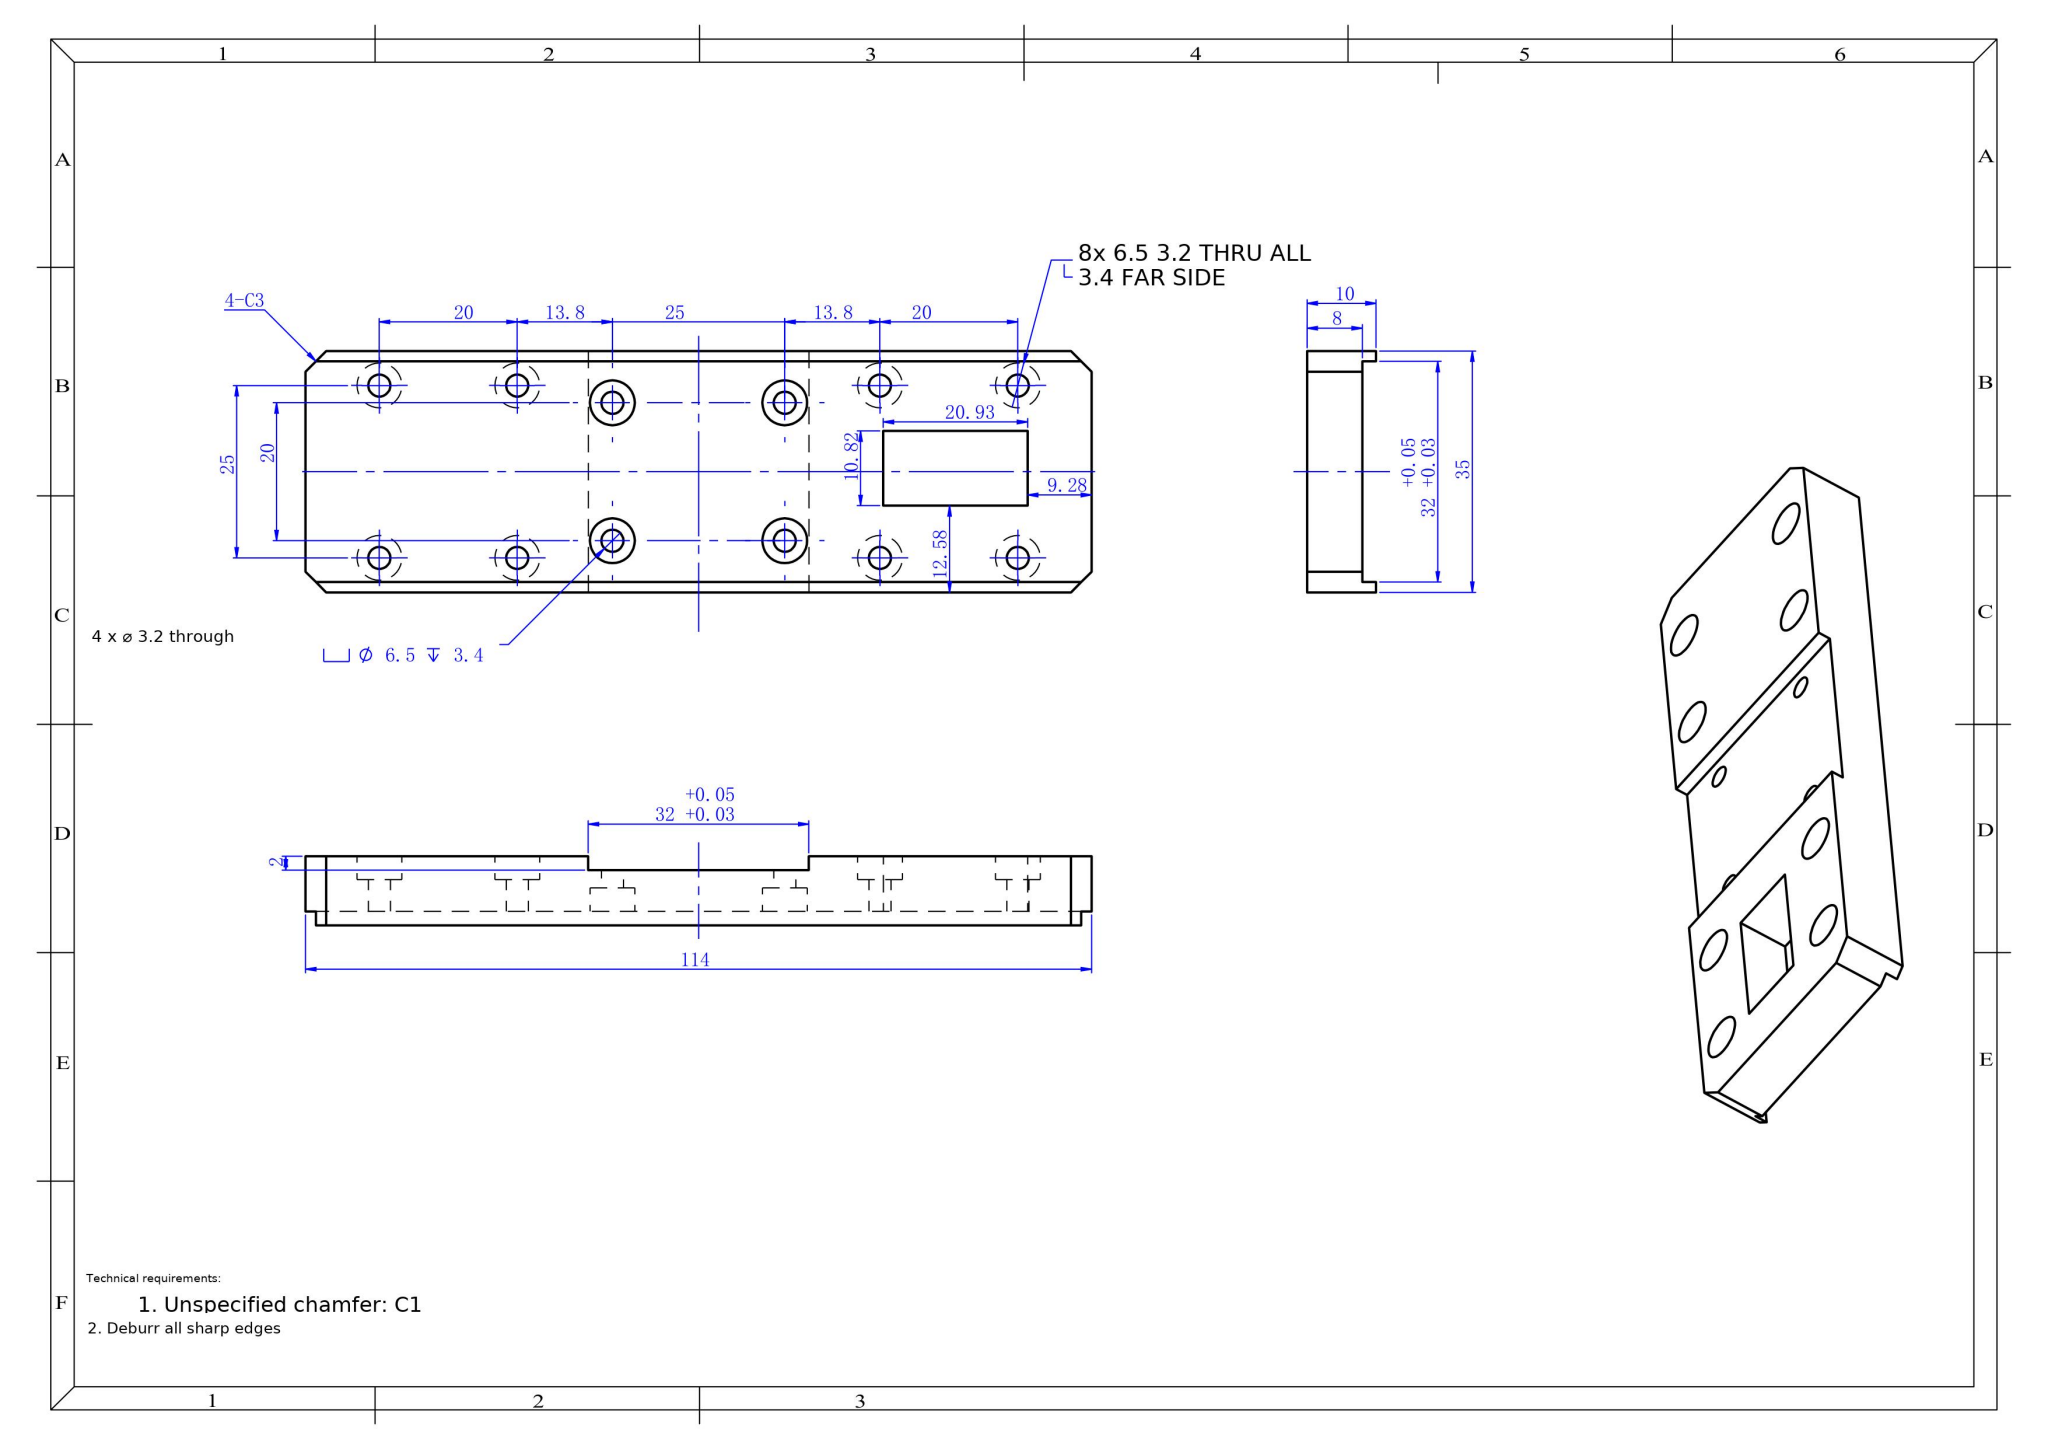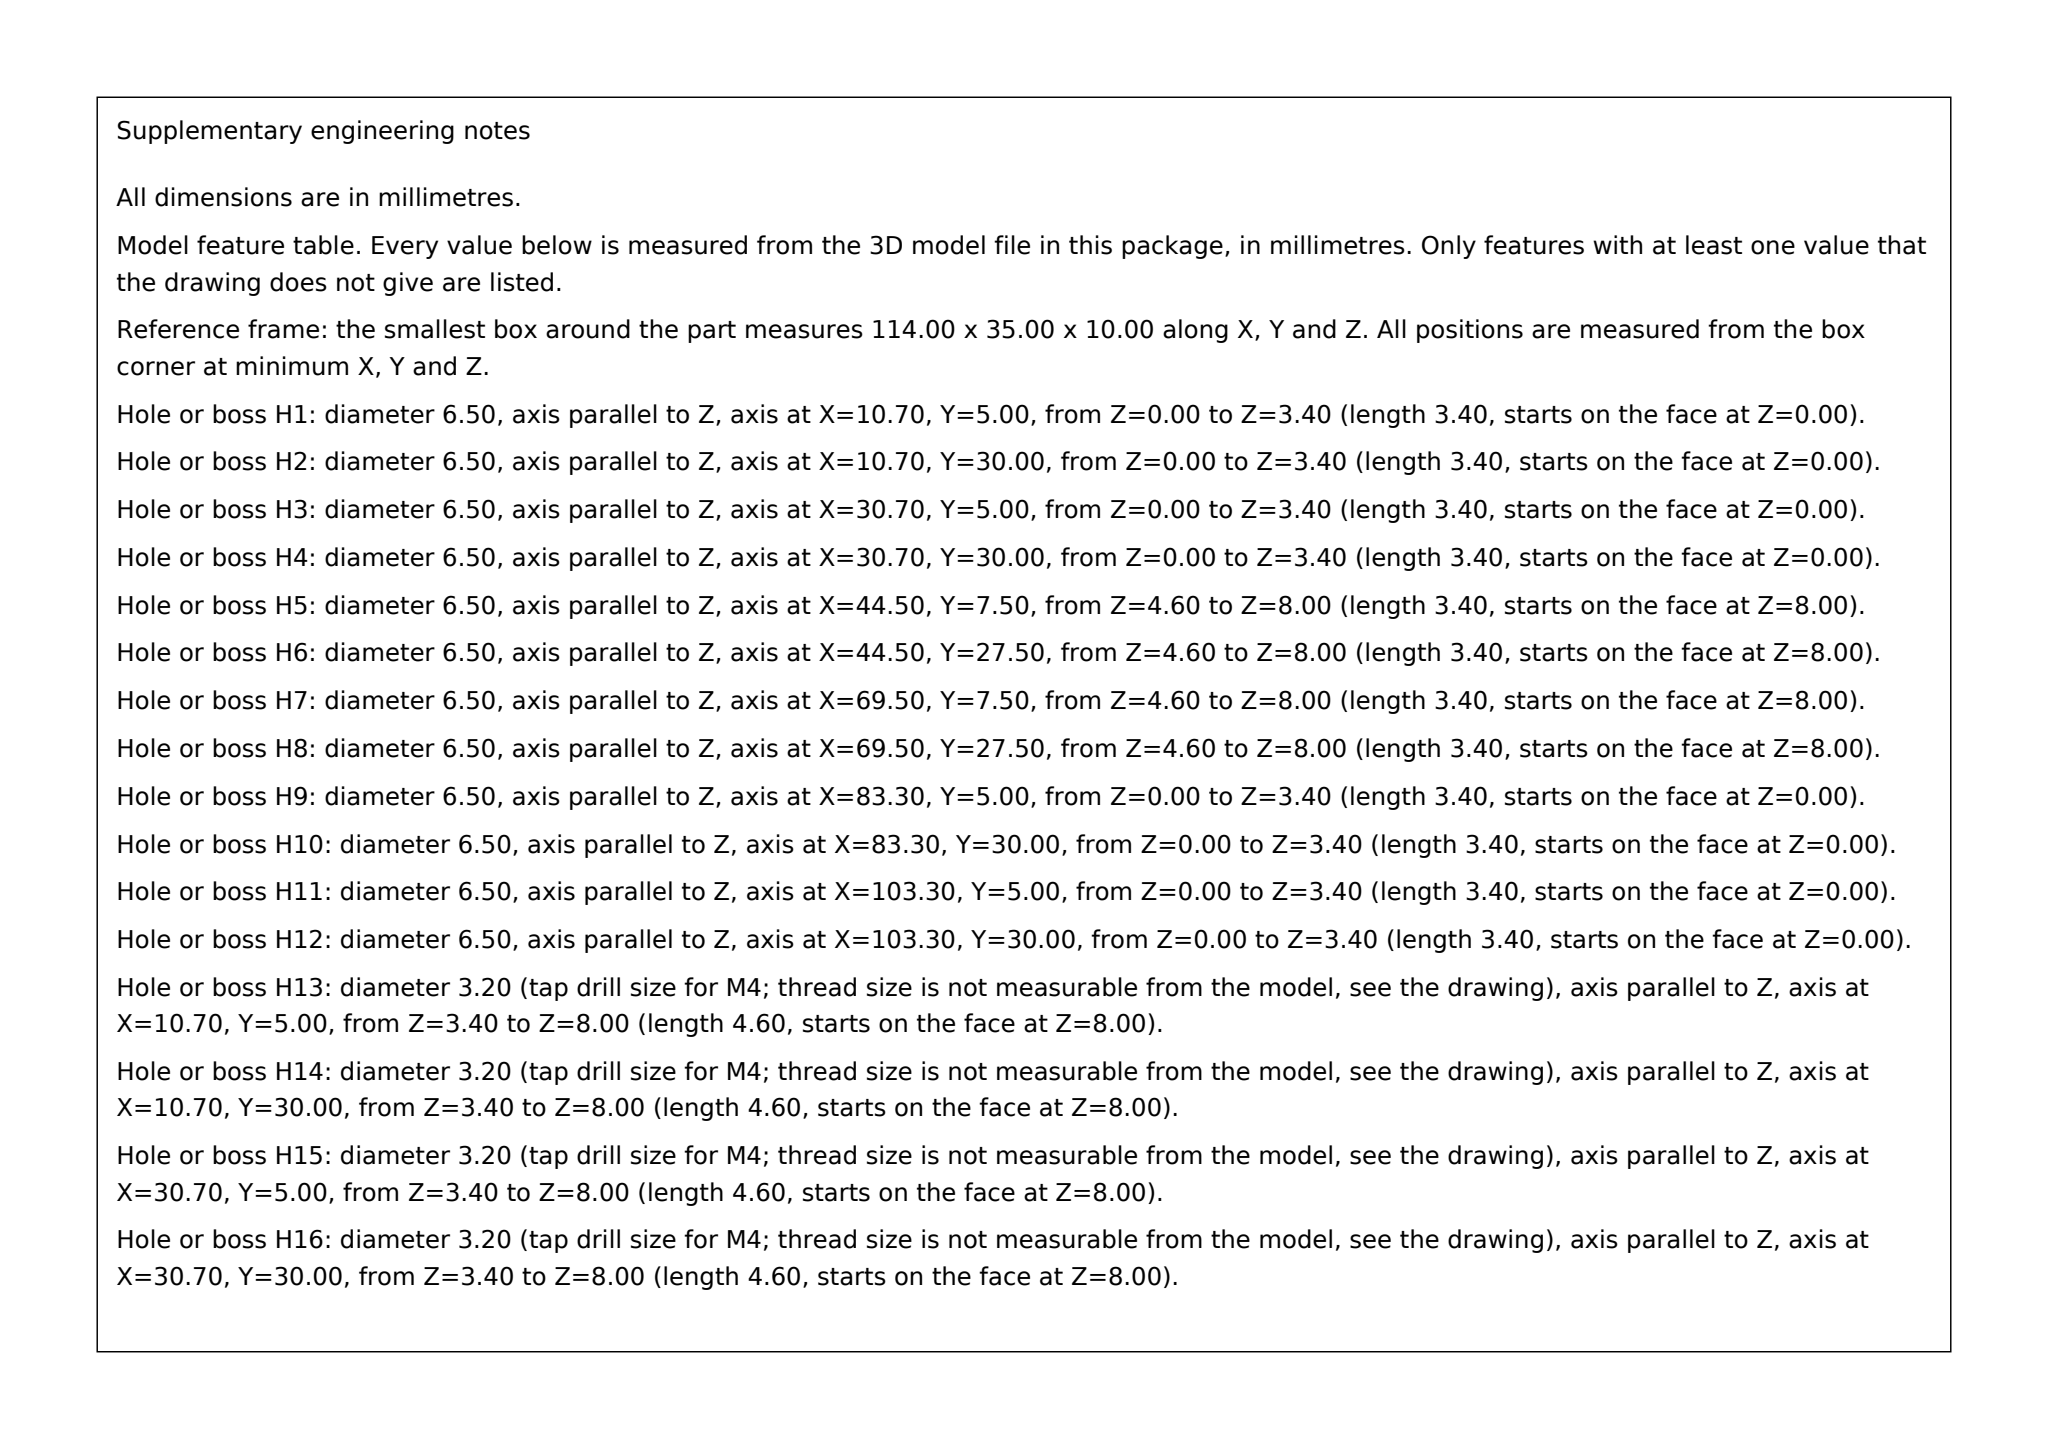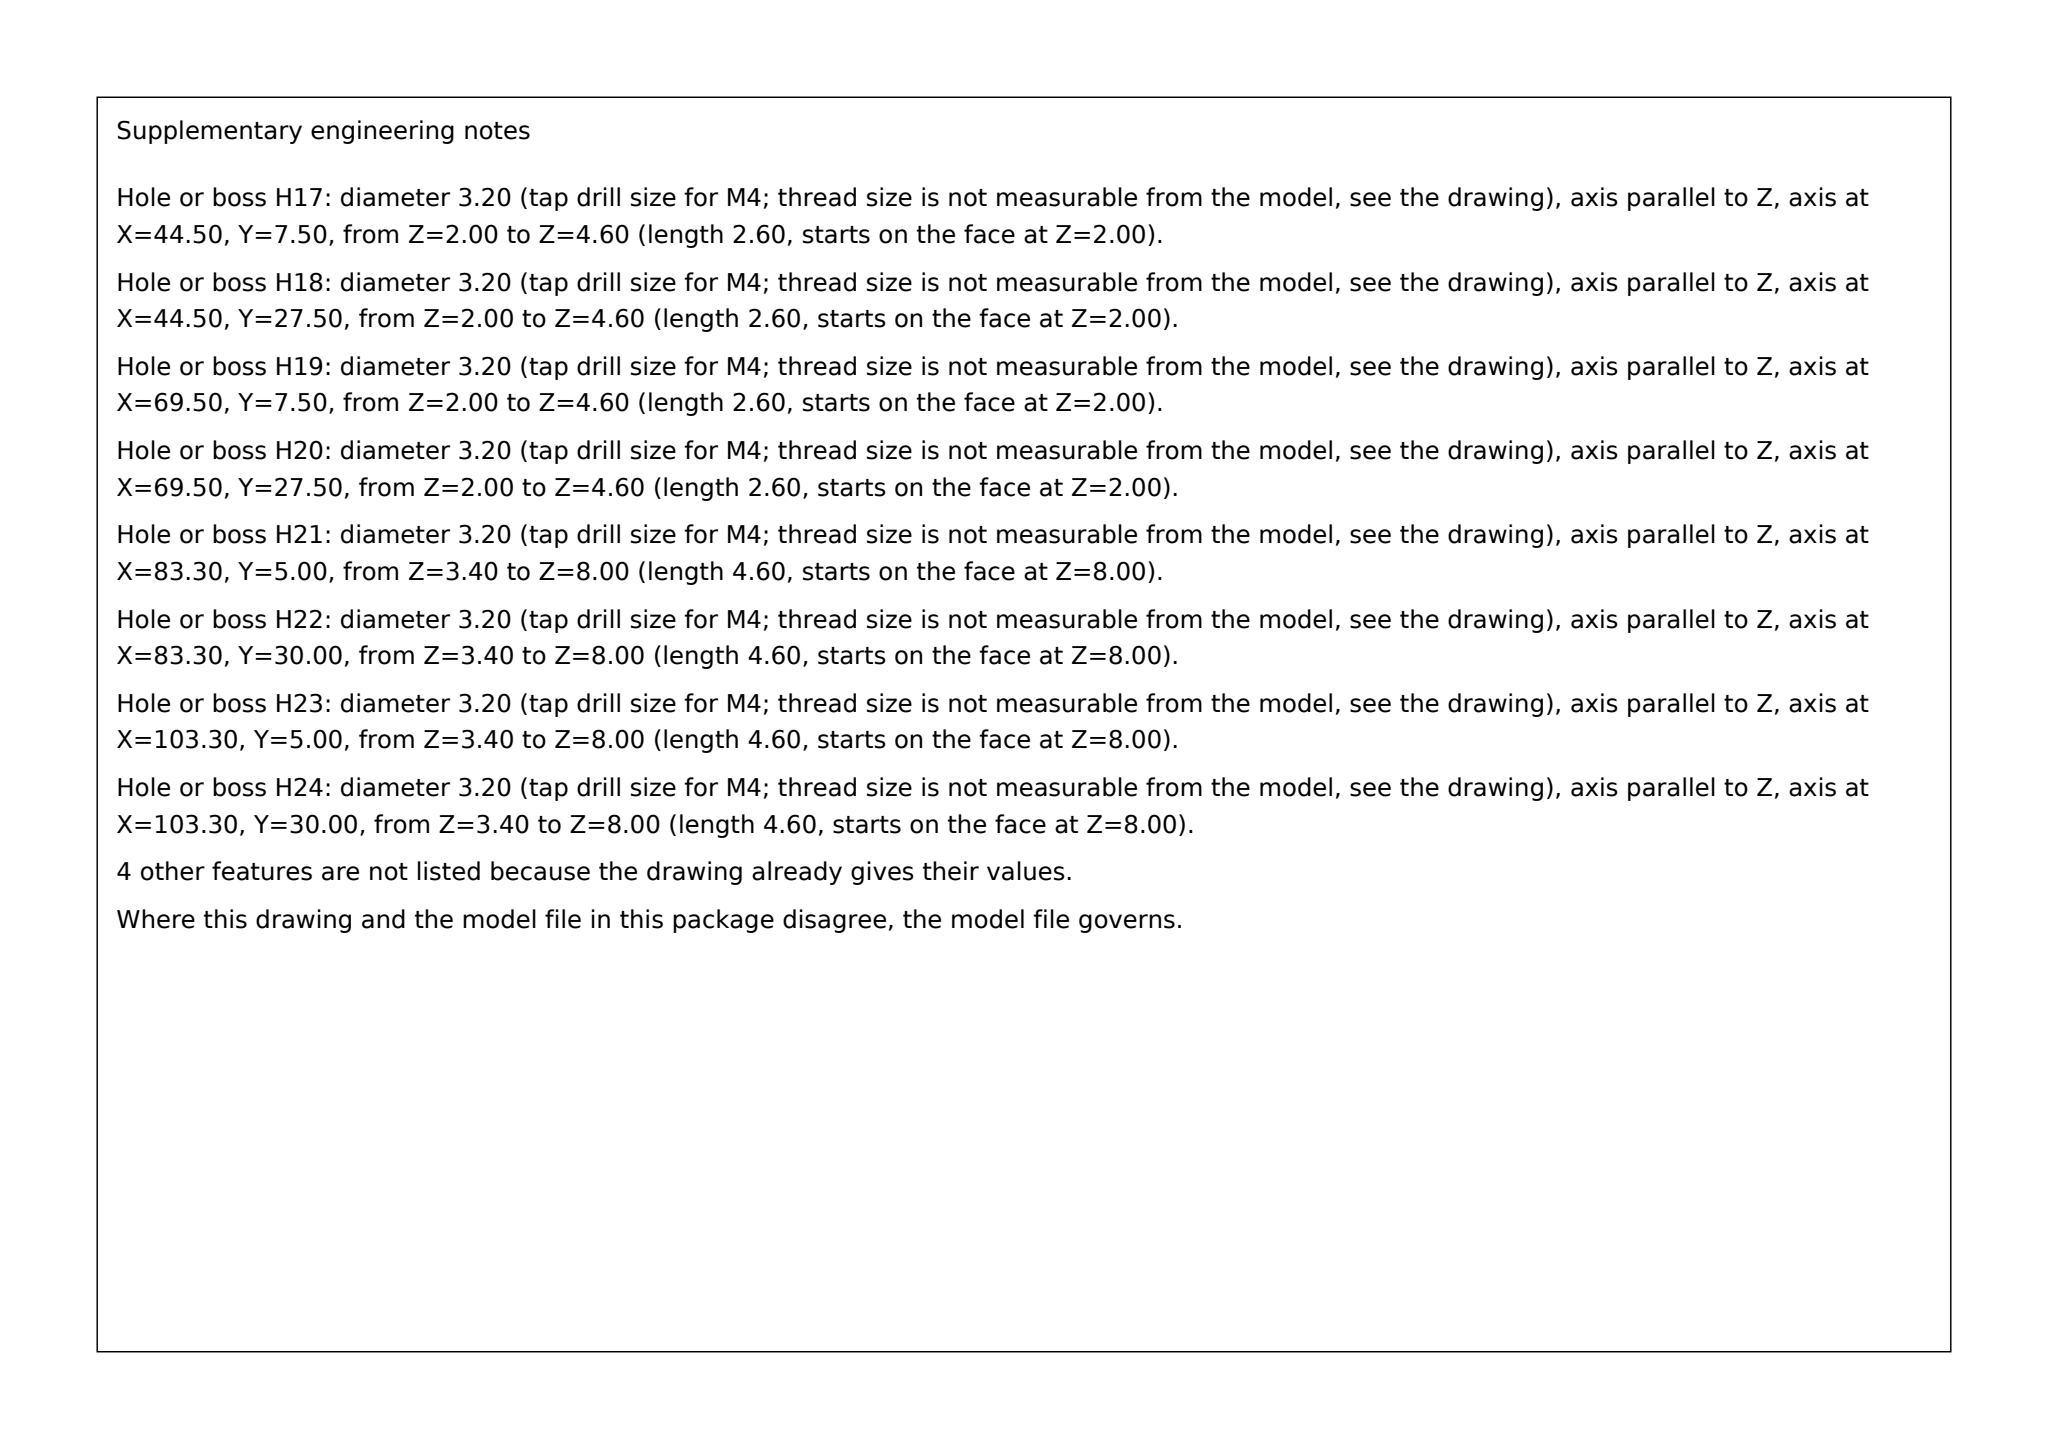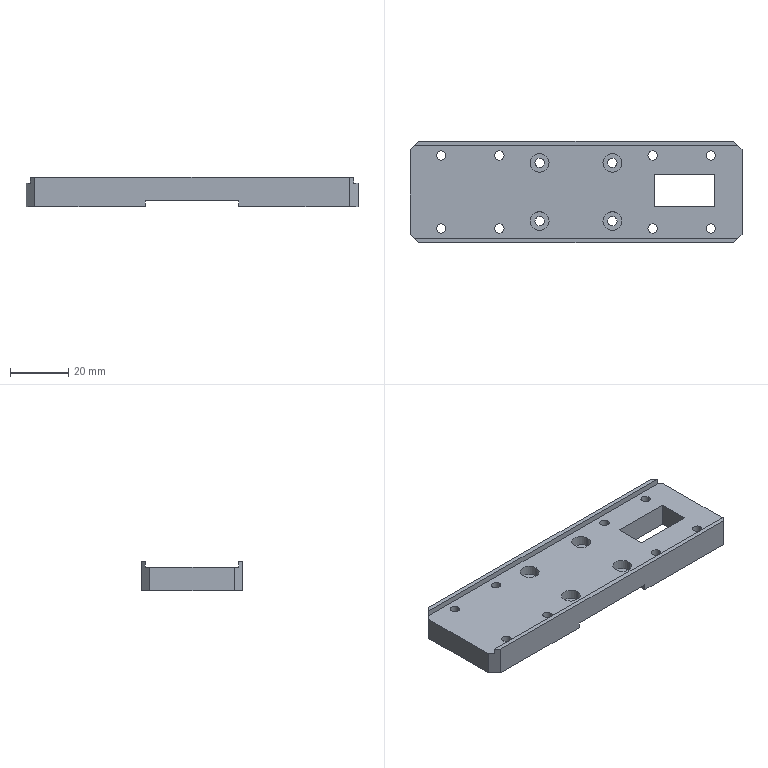Part | SolidWorks | mm | 1 solid | 82 faces | box 114 x 35 x 10 mm | volume 26647 mm3 | cylinder 48 | plane 34 | commonest cylinder face diameters 6.5 x24 3.2 x24
build123d program:
from build123d import *

# Parameters (mm, degrees)
SKETCH1_W                                       = 114
SKETCH1_H                                       = 35
BOSS_EXTRUDE1_DEPTH                             = 10
SKETCH2_W                                       = 2
SKETCH2_H                                       = 32
CUT_EXTRUDE1_DEPTH                              = 118.062
SKETCH3_W                                       = 32
SKETCH3_H                                       = 2
CUT_EXTRUDE2_DEPTH                              = 77.439
M3_HEX_SOCKET_HEAD_CAP_SCREW_CBORE2_D           = 3.2
M3_HEX_SOCKET_HEAD_CAP_SCREW_CBORE2_CBORE_D     = 6.5
M3_HEX_SOCKET_HEAD_CAP_SCREW_CBORE2_CBORE_DEPTH = 3.4
M3_HEX_SOCKET_HEAD_CAP_SCREW_CBORE3_D           = 3.2
M3_HEX_SOCKET_HEAD_CAP_SCREW_CBORE3_CBORE_D     = 6.5
M3_HEX_SOCKET_HEAD_CAP_SCREW_CBORE3_CBORE_DEPTH = 3.4
CHAMFER1_SIZE                                   = 3
CUT_EXTRUDE3_DEPTH                              = 51
CUT_EXTRUDE3_DEPTH_BACK                         = 31
SKETCH12_W                                      = 20.928
SKETCH12_H                                      = 10.825


with BuildPart() as part:
    # Sketch1 → Boss-Extrude1 (new body)
    with BuildSketch(Plane.XY):
        with Locations((10.216, 7.147)):
            Rectangle(SKETCH1_W, SKETCH1_H)
    extrude(amount=BOSS_EXTRUDE1_DEPTH)

    # Sketch2 → Cut-Extrude1 (cut, through all)
    with BuildSketch(Plane(origin=(67.216, 0, 0), x_dir=(0, 0, -1), z_dir=(1, 0, 0))):
        with Locations((-9, 7.147)):
            Rectangle(SKETCH2_W, SKETCH2_H)
    extrude(amount=-CUT_EXTRUDE1_DEPTH, mode=Mode.SUBTRACT)

    # Sketch3 → Cut-Extrude2 (cut, through all)
    with BuildSketch(Plane(origin=(0, 24.647, 0), x_dir=(1, 0, 0), z_dir=(0, 1, 0))):
        with Locations((10.216, -1)):
            Rectangle(SKETCH3_W, SKETCH3_H)
    extrude(amount=-CUT_EXTRUDE2_DEPTH, mode=Mode.SUBTRACT)

    # M3 Hex Socket Head Cap Screw CBORE2 (through all)
    with Locations(Plane.XY.offset(8)):
        with Locations((22.716, 17.147), (22.716, -2.853), (-2.284, -2.853), (-2.284, 17.147)):
            CounterBoreHole(M3_HEX_SOCKET_HEAD_CAP_SCREW_CBORE2_D / 2, M3_HEX_SOCKET_HEAD_CAP_SCREW_CBORE2_CBORE_D / 2, M3_HEX_SOCKET_HEAD_CAP_SCREW_CBORE2_CBORE_DEPTH)

    # M3 Hex Socket Head Cap Screw CBORE3 (through all)
    with Locations(Plane(origin=(0, 0, 0), x_dir=(-1, 0, 0), z_dir=(0, 0, -1))):
        with Locations((-56.516, 19.647), (-36.516, 19.647), (-36.516, -5.353), (-56.516, -5.353)):
            m3_hex_socket_head_cap_screw_cbore3 = CounterBoreHole(M3_HEX_SOCKET_HEAD_CAP_SCREW_CBORE3_D / 2, M3_HEX_SOCKET_HEAD_CAP_SCREW_CBORE3_CBORE_D / 2, M3_HEX_SOCKET_HEAD_CAP_SCREW_CBORE3_CBORE_DEPTH)

    # Mirror2: M3 Hex Socket Head Cap Screw CBORE3 across plane
    add(m3_hex_socket_head_cap_screw_cbore3.mirror(Plane(origin=(10.216, 0, 0), x_dir=(0, 0, 1), z_dir=(1, 0, 0))), mode=Mode.SUBTRACT)

    # Chamfer1
    chamfer1_edges = [part.edges().sort_by_distance(p)[0] for p in [
        (-46.784, -10.353, 5),
        (-46.784, 24.647, 5),
        (67.216, -10.353, 5),
        (67.216, 24.647, 5),
    ]]
    chamfer(chamfer1_edges, length=CHAMFER1_SIZE)

    # Sketch12 → Cut-Extrude3 (cut, two sides: drawn at the far end of the back side and taken through both)
    with BuildSketch(Plane(origin=(0, 0, 2), x_dir=(-1, 0, 0), z_dir=(0, 0, -1)).offset(-CUT_EXTRUDE3_DEPTH_BACK)):
        with Locations((-47.47, 7.643)):
            Rectangle(SKETCH12_W, SKETCH12_H)
    extrude(amount=CUT_EXTRUDE3_DEPTH + CUT_EXTRUDE3_DEPTH_BACK, mode=Mode.SUBTRACT)


solid = part.part